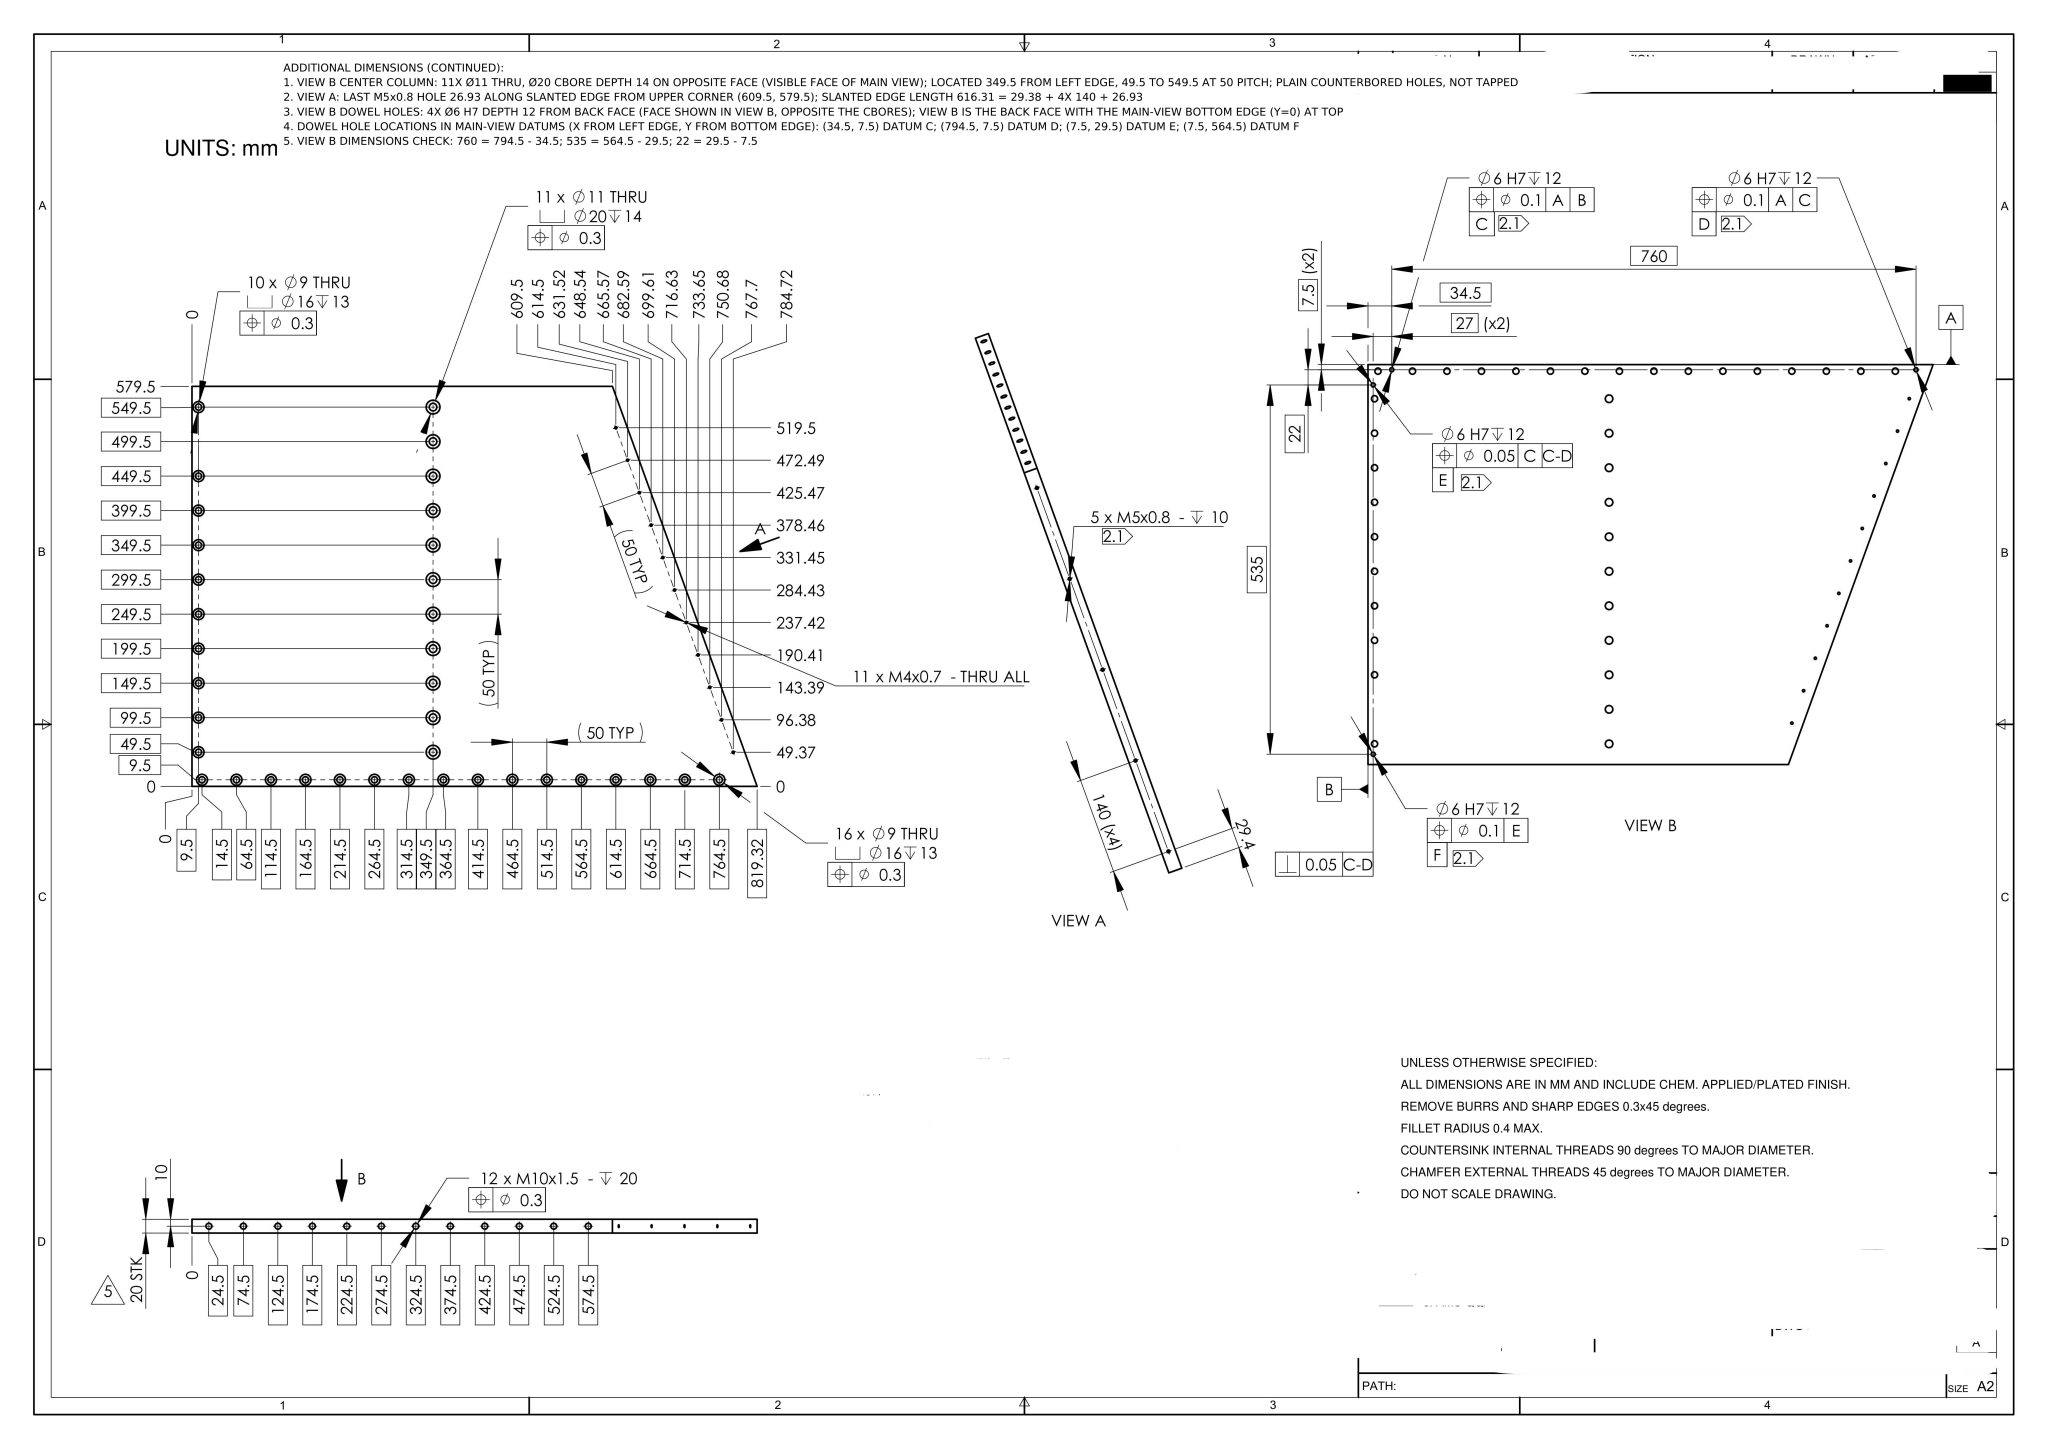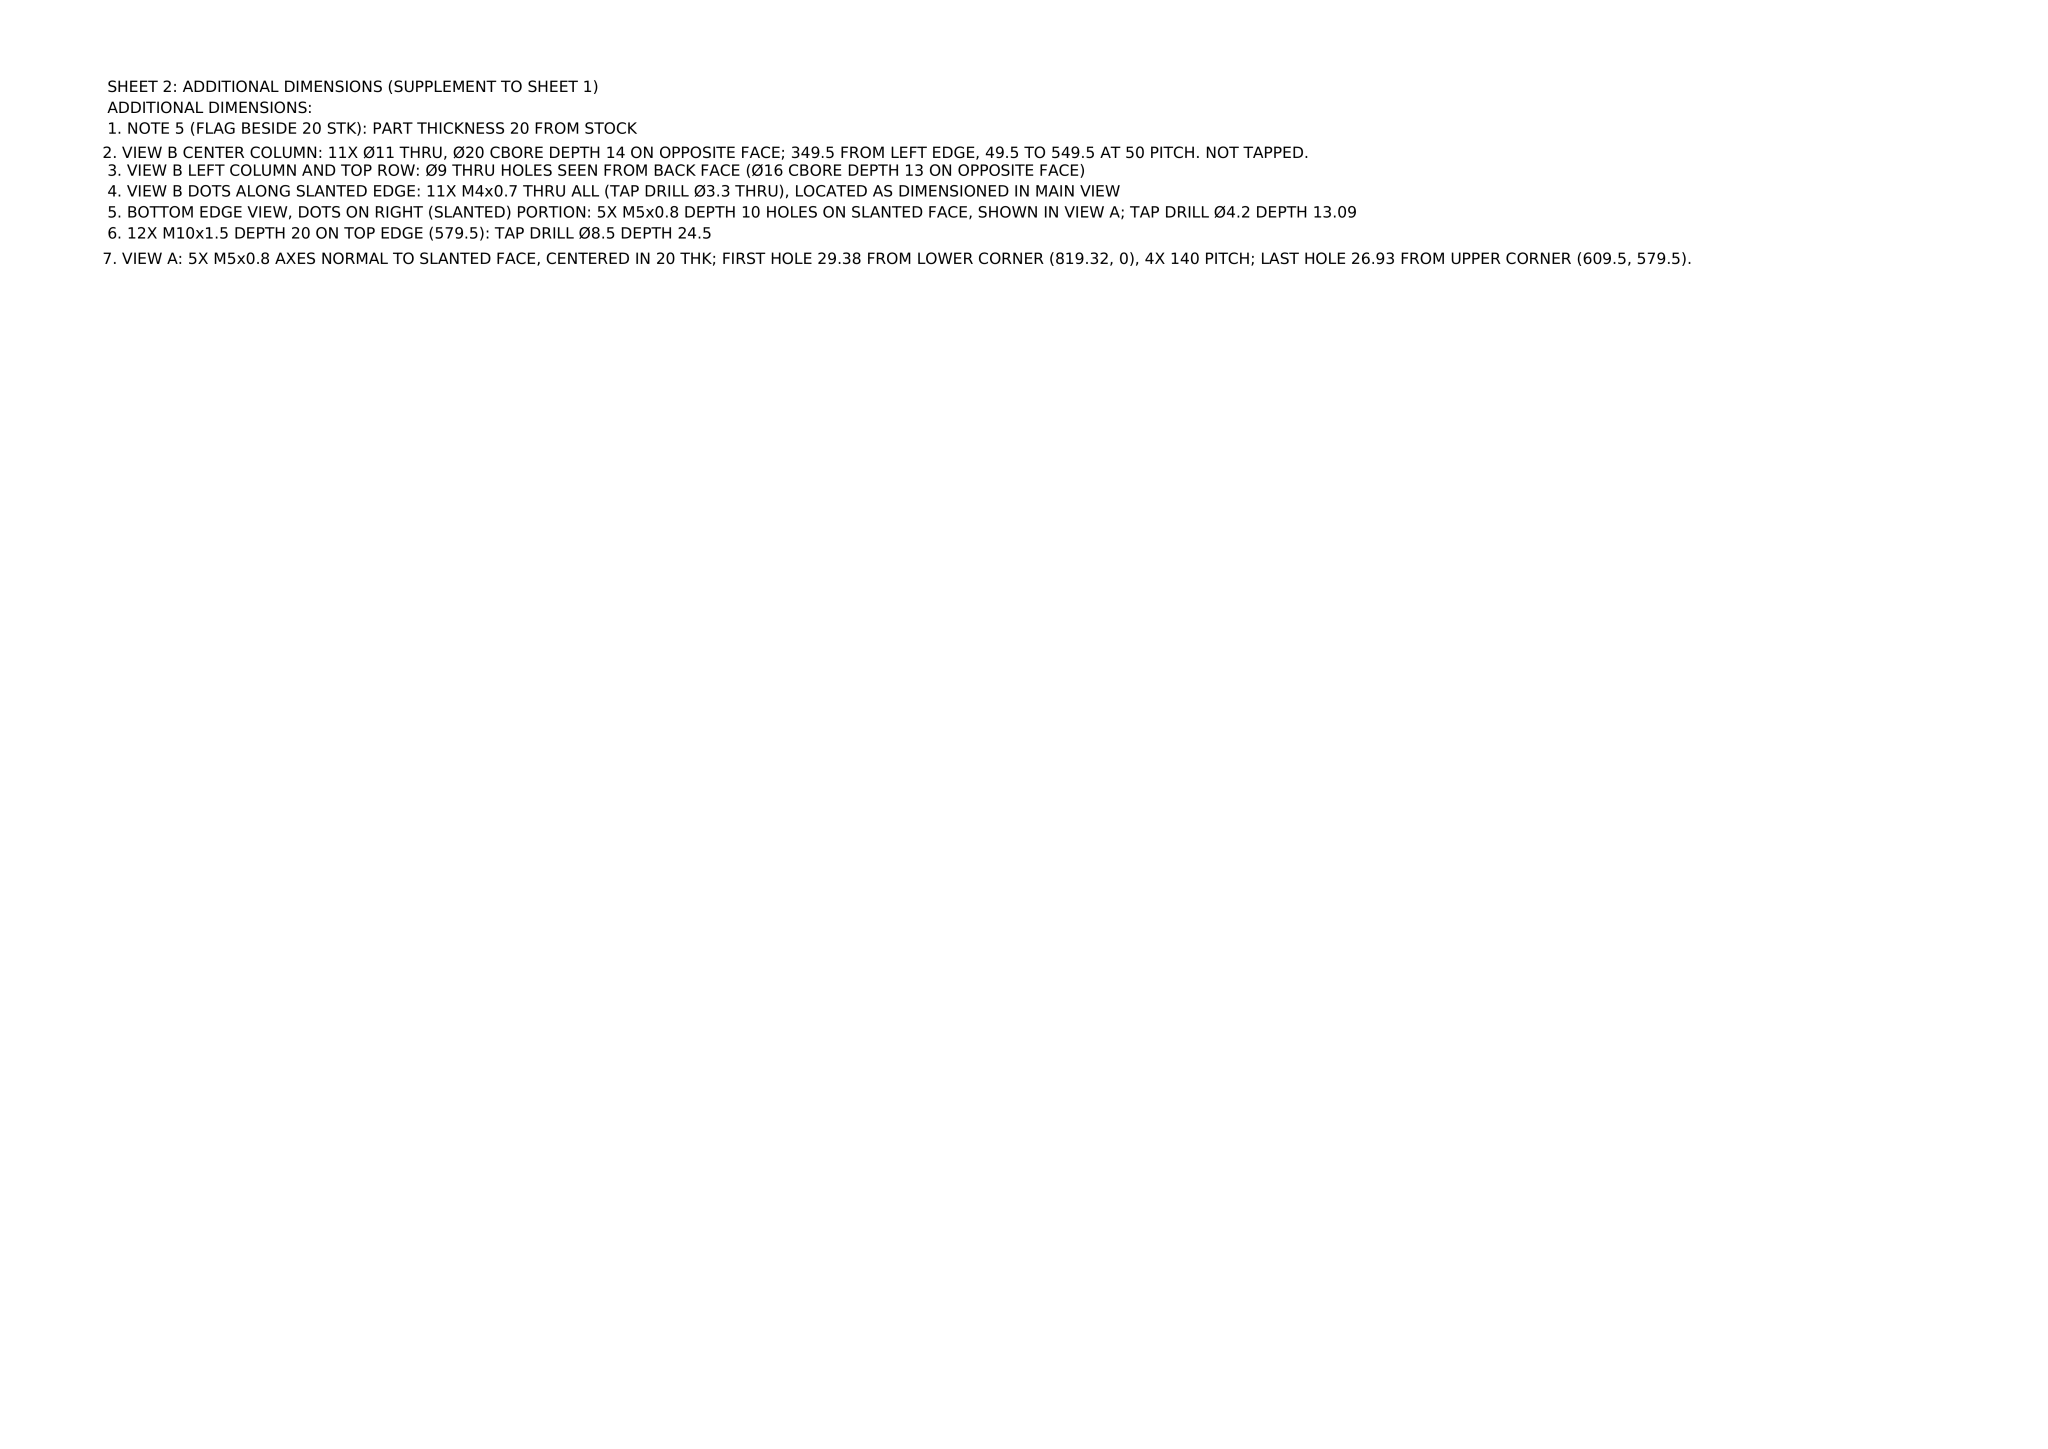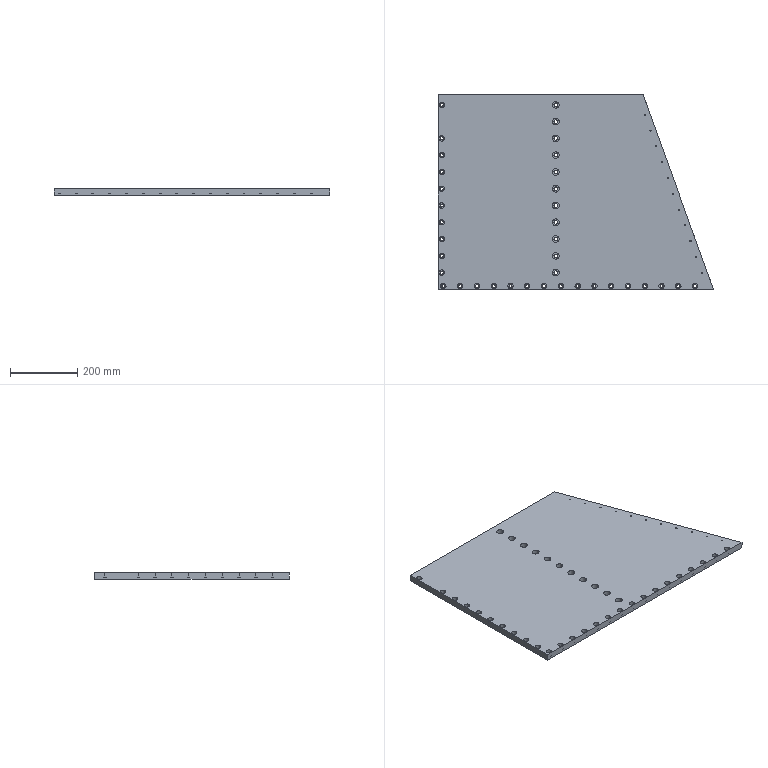Part | NX | mm | 1 solid | 297 faces | box 819.32 x 579.5 x 20 mm | volume 8124358 mm3 | cylinder 212 | plane 43 | cone 42 | commonest cylinder face diameters 16 x52 9 x52 8.5 x24 20 x22 3.3 x22 11 x22 4.2 x10 6 x8